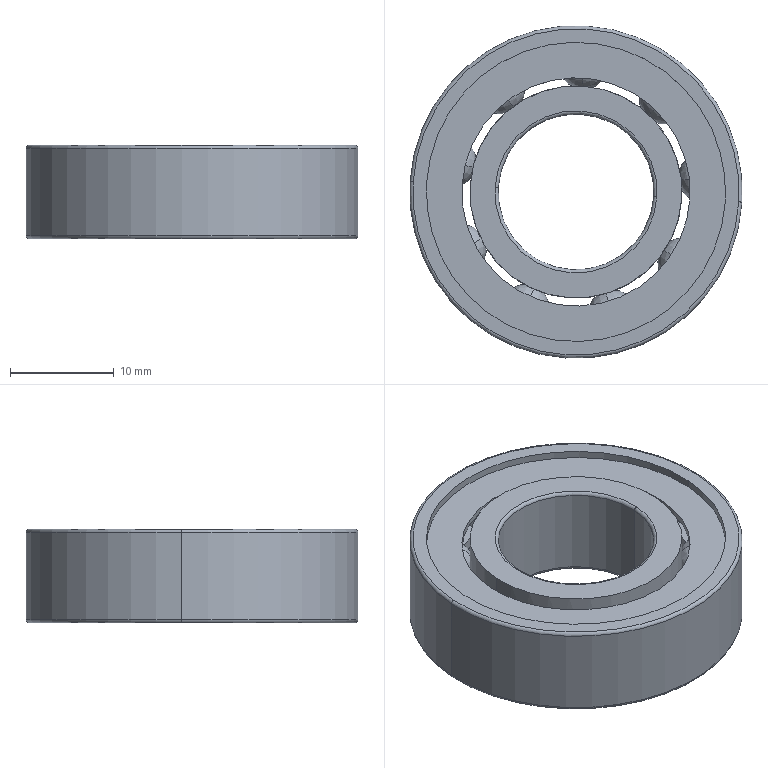Component | SolidWorks | 04DeepGrooveBallBearing6002-2Z-2 | 1 solid | 160 faces | volume 3407 mm3 | sphere 72 | torus 38 | plane 26 | cylinder 24 | commonest cylinder face diameters 28.8 x8 20.4 x4 21.971 x2 15 x2 32 x2 28.5 x2 25.91 x2 23.29 x2